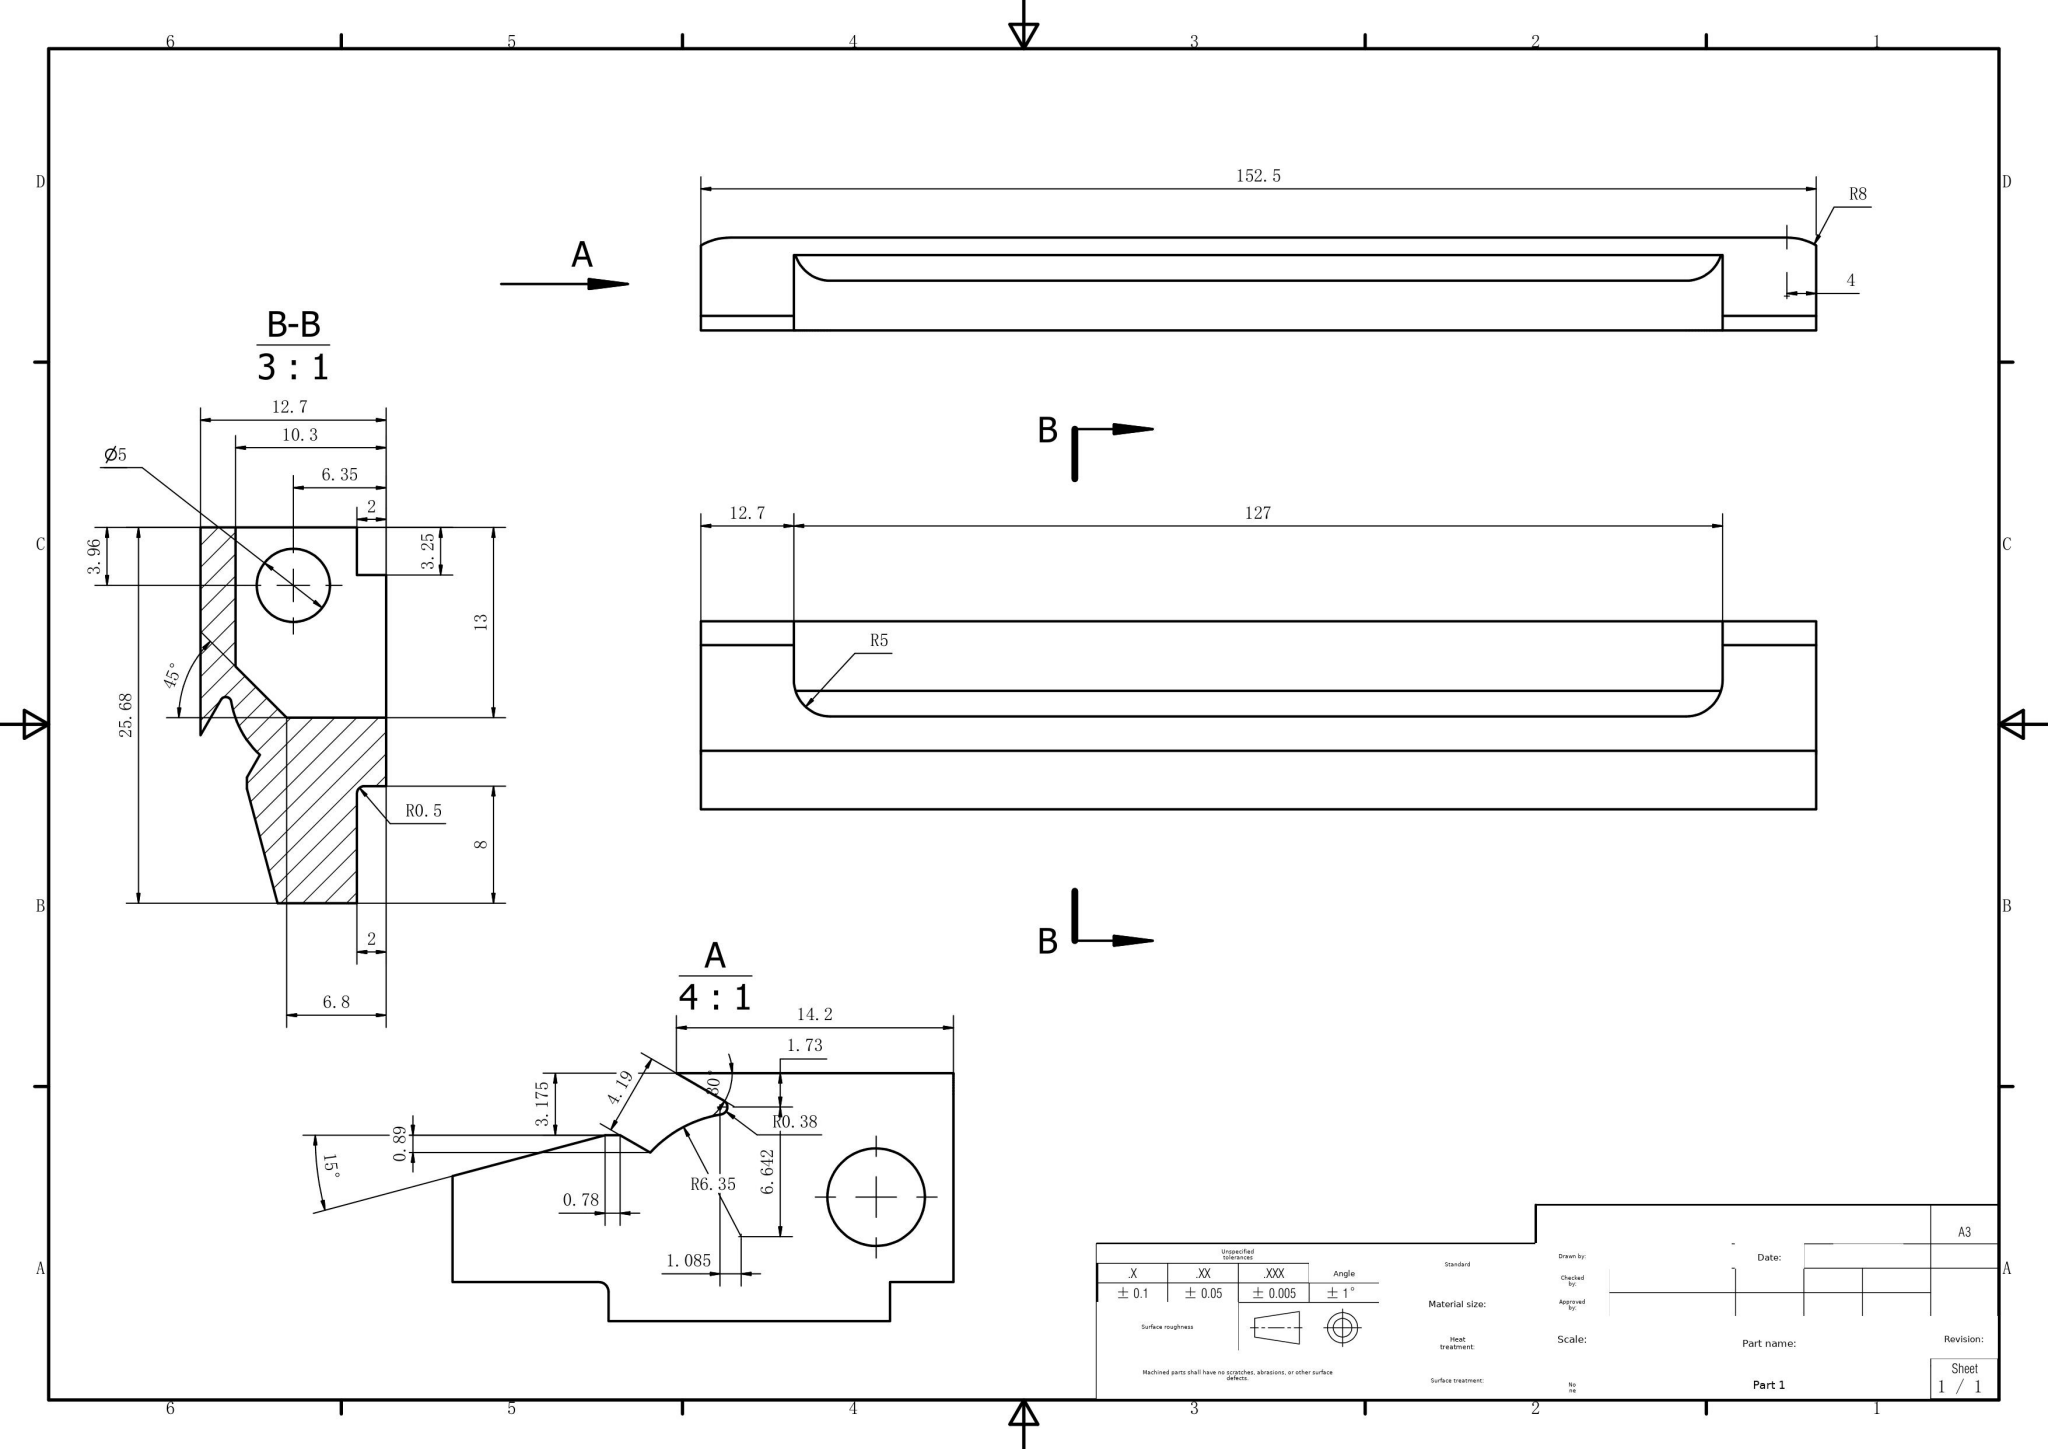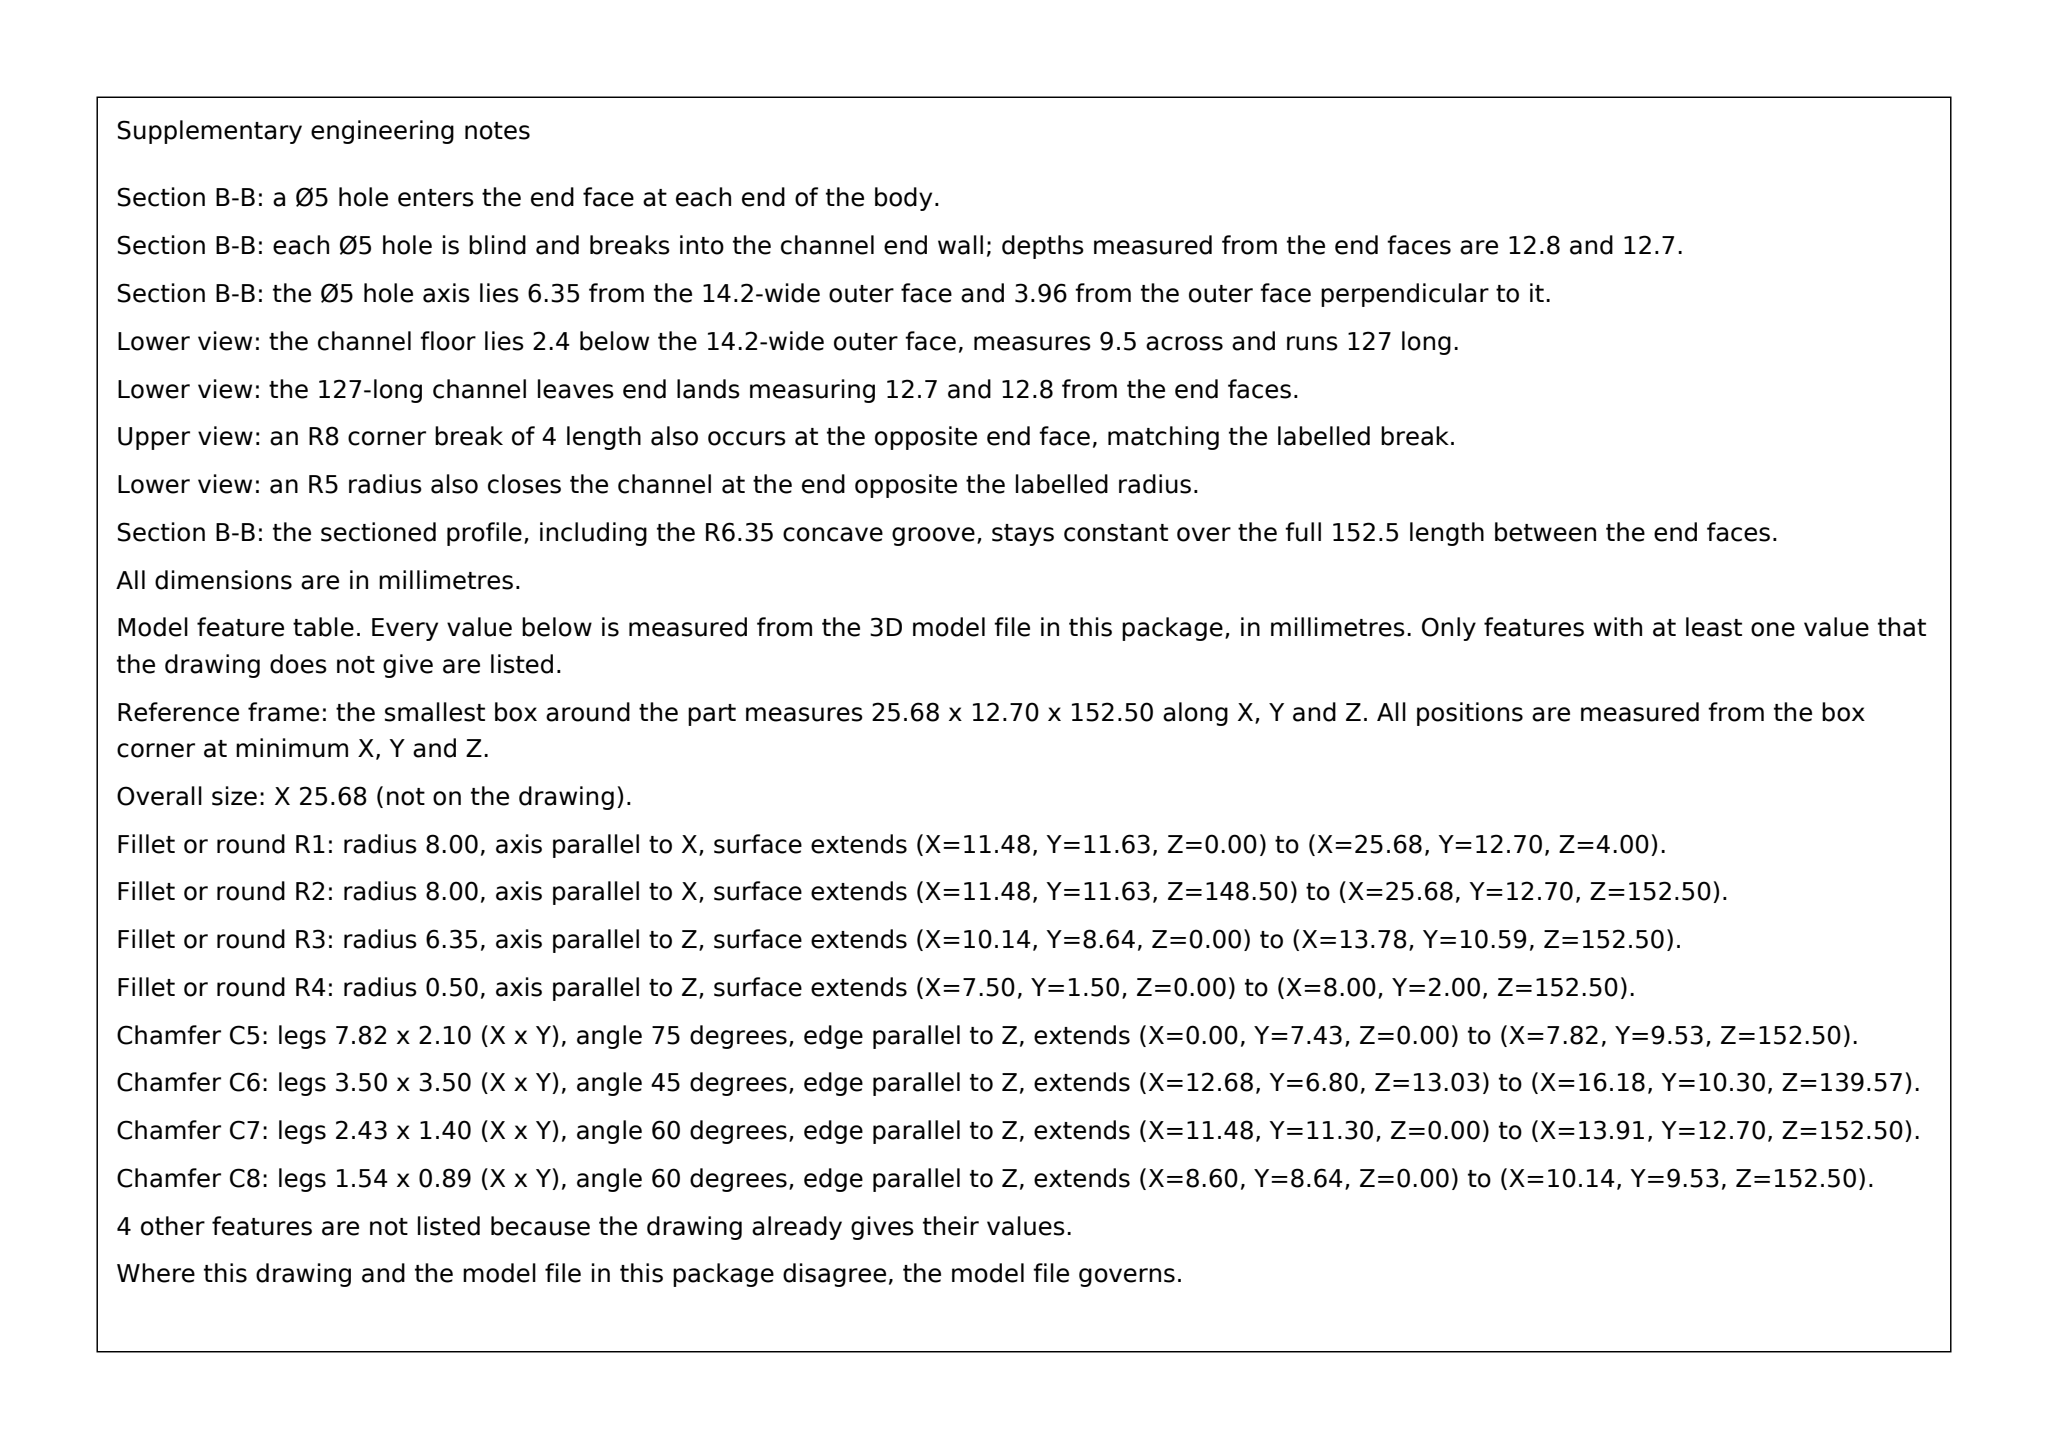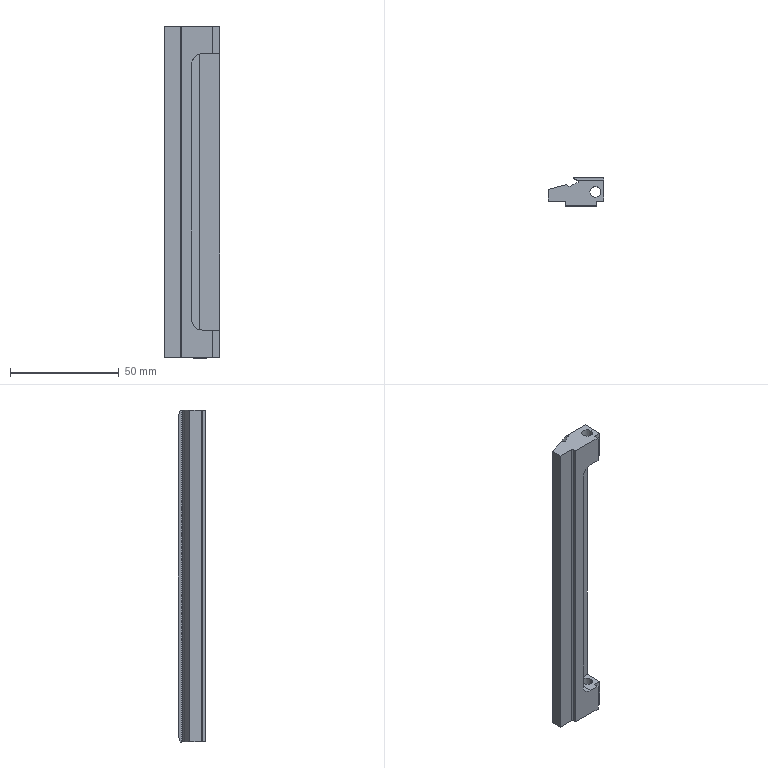Part | SolidWorks | mm | 1 solid | 32 faces | box 25.68 x 12.7 x 152.5 mm | volume 22834 mm3 | plane 21 | cylinder 11 | commonest cylinder face diameters 5 x4 16 x2 10 x2 0.76 x1 12.7 x1 1 x1
Drawing notes:
127 GROOVE: 12.8 FROM LH END FACE, 12.7 FROM RH END FACE | from the solid: z planes at 12.8 and 139.8 on 152.5 length (bbox z=152.5)
4 STEP & R8 2X, BOTH ENDS; R8 CL 4 FROM EACH END FACE | from the solid: Ø16 (R8) x-axis cyls at z=4.0 and z=148.5, 152.5-148.5=4
R5 2X, TANGENT AT 12.8 & 139.8 FROM LH END FACE | from the solid: Ø10 (R5) y-axis cyls at z=17.8 and z=134.8, len 10.3
2X Ø5 THRU AXIAL IN END TABS: 12.8 LH, 12.7 RH | from the solid: Ø5 z-axis cyls at x21.72/y6.35, lengths 12.8 (z0-12.8) and 12.7 (z139.8-152.5)
SECT B-B CUT IN LH END TAB, BTWN 0 AND 12.8 FROM END FACE | from the solid: Ø5 bore and tab section exist only z=0-12.8 and z=139.8-152.5